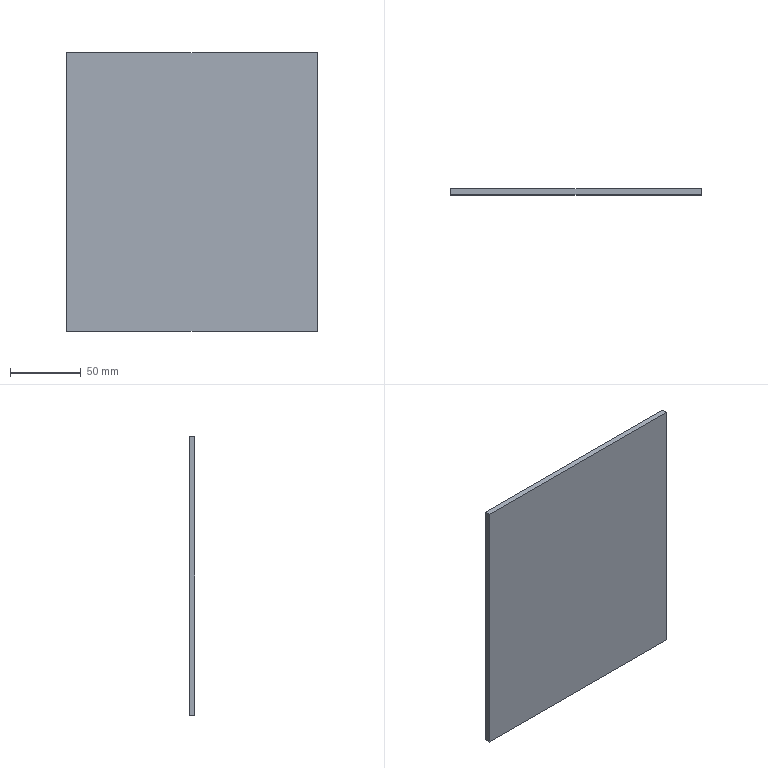Component | SolidWorks | Cover1-5XG1-1 | 1 solid | 6 faces | box 177 x 4 x 197 mm | volume 139476 mm3 | plane 6
build123d program:
from build123d import *

# Parameters (mm, degrees)
SKETCH3_W           = 177
SKETCH3_H           = 197
BOSS_EXTRUDE1_DEPTH = 4


with BuildPart() as part:
    # Sketch3 → Boss-Extrude1 (new body)
    with BuildSketch(Plane.XY):
        Rectangle(SKETCH3_W, SKETCH3_H)
    extrude(amount=BOSS_EXTRUDE1_DEPTH)


solid = part.part

# Placed as in the assembly
solid = solid.moved(Location((0, -154.8, 130), (90, 0, 0)))
STEP:
#1=COLOUR_RGB('',0.7922,0.8196,0.9333);
#2=FILL_AREA_STYLE_COLOUR('',#1);
#3=FILL_AREA_STYLE('',(#2));
#4=SURFACE_STYLE_FILL_AREA(#3);
#5=SURFACE_SIDE_STYLE('',(#4));
#6=SURFACE_STYLE_USAGE(.BOTH.,#5);
#7=PRESENTATION_STYLE_ASSIGNMENT((#6));
#8=CARTESIAN_POINT('',(-3.484,-6.252,1.24));
#9=VERTEX_POINT('',#8);
#10=CARTESIAN_POINT('',(-3.484,-6.252,8.996));
#11=VERTEX_POINT('',#10);
#12=CARTESIAN_POINT('',(-3.484,-6.252,1.24));
#13=DIRECTION('',(-0.,-0.,1.));
#14=VECTOR('',#13,39.37);
#15=LINE('',#12,#14);
#16=EDGE_CURVE('',#9,#11,#15,.T.);
#17=ORIENTED_EDGE('',*,*,#16,.T.);
#18=CARTESIAN_POINT('',(-3.484,-6.094,8.996));
#19=VERTEX_POINT('',#18);
#20=CARTESIAN_POINT('',(-3.484,-6.094,8.996));
#21=DIRECTION('',(-0.,-1.,-0.));
#22=VECTOR('',#21,39.37);
#23=LINE('',#20,#22);
#24=EDGE_CURVE('',#19,#11,#23,.T.);
#25=ORIENTED_EDGE('',*,*,#24,.F.);
#26=CARTESIAN_POINT('',(-3.484,-6.094,1.24));
#27=VERTEX_POINT('',#26);
#28=CARTESIAN_POINT('',(-3.484,-6.094,1.24));
#29=DIRECTION('',(-0.,-0.,1.));
#30=VECTOR('',#29,39.37);
#31=LINE('',#28,#30);
#32=EDGE_CURVE('',#27,#19,#31,.T.);
#33=ORIENTED_EDGE('',*,*,#32,.F.);
#34=CARTESIAN_POINT('',(-3.484,-6.094,1.24));
#35=DIRECTION('',(-0.,-1.,-0.));
#36=VECTOR('',#35,39.37);
#37=LINE('',#34,#36);
#38=EDGE_CURVE('',#27,#9,#37,.T.);
#39=ORIENTED_EDGE('',*,*,#38,.T.);
#40=EDGE_LOOP('',(#17,#25,#33,#39));
#41=FACE_OUTER_BOUND('',#40,.T.);
#42=CARTESIAN_POINT('',(-3.484,-6.094,1.24));
#43=DIRECTION('',(1.,-0.,0.));
#44=DIRECTION('',(-0.,-1.,-0.));
#45=AXIS2_PLACEMENT_3D('',#42,#43,#44);
#46=PLANE('',#45);
#47=ADVANCED_FACE('',(#41),#46,.F.);
#48=CARTESIAN_POINT('',(3.484,-6.252,8.996));
#49=VERTEX_POINT('',#48);
#50=CARTESIAN_POINT('',(-3.484,-6.252,8.996));
#51=DIRECTION('',(1.,-0.,0.));
#52=VECTOR('',#51,39.37);
#53=LINE('',#50,#52);
#54=EDGE_CURVE('',#11,#49,#53,.T.);
#55=ORIENTED_EDGE('',*,*,#54,.T.);
#56=CARTESIAN_POINT('',(3.484,-6.094,8.996));
#57=VERTEX_POINT('',#56);
#58=CARTESIAN_POINT('',(3.484,-6.094,8.996));
#59=DIRECTION('',(-0.,-1.,-0.));
#60=VECTOR('',#59,39.37);
#61=LINE('',#58,#60);
#62=EDGE_CURVE('',#57,#49,#61,.T.);
#63=ORIENTED_EDGE('',*,*,#62,.F.);
#64=CARTESIAN_POINT('',(-3.484,-6.094,8.996));
#65=DIRECTION('',(1.,-0.,0.));
#66=VECTOR('',#65,39.37);
#67=LINE('',#64,#66);
#68=EDGE_CURVE('',#19,#57,#67,.T.);
#69=ORIENTED_EDGE('',*,*,#68,.F.);
#70=ORIENTED_EDGE('',*,*,#24,.T.);
#71=EDGE_LOOP('',(#55,#63,#69,#70));
#72=FACE_OUTER_BOUND('',#71,.T.);
#73=CARTESIAN_POINT('',(-3.484,-6.094,8.996));
#74=DIRECTION('',(0.,0.,-1.));
#75=DIRECTION('',(0.,1.,0.));
#76=AXIS2_PLACEMENT_3D('',#73,#74,#75);
#77=PLANE('',#76);
#78=ADVANCED_FACE('',(#72),#77,.F.);
#79=CARTESIAN_POINT('',(3.484,-6.252,1.24));
#80=VERTEX_POINT('',#79);
#81=CARTESIAN_POINT('',(3.484,-6.252,1.24));
#82=DIRECTION('',(0.,0.,-1.));
#83=VECTOR('',#82,39.37);
#84=LINE('',#81,#83);
#85=EDGE_CURVE('',#49,#80,#84,.T.);
#86=ORIENTED_EDGE('',*,*,#85,.T.);
#87=CARTESIAN_POINT('',(3.484,-6.094,1.24));
#88=VERTEX_POINT('',#87);
#89=CARTESIAN_POINT('',(3.484,-6.094,1.24));
#90=DIRECTION('',(-0.,-1.,-0.));
#91=VECTOR('',#90,39.37);
#92=LINE('',#89,#91);
#93=EDGE_CURVE('',#88,#80,#92,.T.);
#94=ORIENTED_EDGE('',*,*,#93,.F.);
#95=CARTESIAN_POINT('',(3.484,-6.094,1.24));
#96=DIRECTION('',(0.,0.,-1.));
#97=VECTOR('',#96,39.37);
#98=LINE('',#95,#97);
#99=EDGE_CURVE('',#57,#88,#98,.T.);
#100=ORIENTED_EDGE('',*,*,#99,.F.);
#101=ORIENTED_EDGE('',*,*,#62,.T.);
#102=EDGE_LOOP('',(#86,#94,#100,#101));
#103=FACE_OUTER_BOUND('',#102,.T.);
#104=CARTESIAN_POINT('',(3.484,-6.094,1.24));
#105=DIRECTION('',(-1.,0.,-0.));
#106=DIRECTION('',(0.,1.,0.));
#107=AXIS2_PLACEMENT_3D('',#104,#105,#106);
#108=PLANE('',#107);
#109=ADVANCED_FACE('',(#103),#108,.F.);
#110=CARTESIAN_POINT('',(-3.484,-6.252,1.24));
#111=DIRECTION('',(-1.,0.,-0.));
#112=VECTOR('',#111,39.37);
#113=LINE('',#110,#112);
#114=EDGE_CURVE('',#80,#9,#113,.T.);
#115=ORIENTED_EDGE('',*,*,#114,.T.);
#116=ORIENTED_EDGE('',*,*,#38,.F.);
#117=CARTESIAN_POINT('',(-3.484,-6.094,1.24));
#118=DIRECTION('',(-1.,0.,-0.));
#119=VECTOR('',#118,39.37);
#120=LINE('',#117,#119);
#121=EDGE_CURVE('',#88,#27,#120,.T.);
#122=ORIENTED_EDGE('',*,*,#121,.F.);
#123=ORIENTED_EDGE('',*,*,#93,.T.);
#124=EDGE_LOOP('',(#115,#116,#122,#123));
#125=FACE_OUTER_BOUND('',#124,.T.);
#126=CARTESIAN_POINT('',(-3.484,-6.094,1.24));
#127=DIRECTION('',(-0.,-0.,1.));
#128=DIRECTION('',(-0.,-1.,-0.));
#129=AXIS2_PLACEMENT_3D('',#126,#127,#128);
#130=PLANE('',#129);
#131=ADVANCED_FACE('',(#125),#130,.F.);
#132=ORIENTED_EDGE('',*,*,#32,.T.);
#133=ORIENTED_EDGE('',*,*,#68,.T.);
#134=ORIENTED_EDGE('',*,*,#99,.T.);
#135=ORIENTED_EDGE('',*,*,#121,.T.);
#136=EDGE_LOOP('',(#132,#133,#134,#135));
#137=FACE_OUTER_BOUND('',#136,.T.);
#138=CARTESIAN_POINT('',(0.,-6.094,5.118));
#139=DIRECTION('',(0.,1.,0.));
#140=DIRECTION('',(1.,-0.,0.));
#141=AXIS2_PLACEMENT_3D('',#138,#139,#140);
#142=PLANE('',#141);
#143=ADVANCED_FACE('',(#137),#142,.T.);
#144=ORIENTED_EDGE('',*,*,#16,.F.);
#145=ORIENTED_EDGE('',*,*,#114,.F.);
#146=ORIENTED_EDGE('',*,*,#85,.F.);
#147=ORIENTED_EDGE('',*,*,#54,.F.);
#148=EDGE_LOOP('',(#144,#145,#146,#147));
#149=FACE_OUTER_BOUND('',#148,.T.);
#150=CARTESIAN_POINT('',(0.,-6.252,5.118));
#151=DIRECTION('',(0.,1.,0.));
#152=DIRECTION('',(1.,-0.,0.));
#153=AXIS2_PLACEMENT_3D('',#150,#151,#152);
#154=PLANE('',#153);
#155=ADVANCED_FACE('',(#149),#154,.F.);
#156=CLOSED_SHELL('',(#47,#78,#109,#131,#143,#155));
#157=MANIFOLD_SOLID_BREP('',#156);
#158=STYLED_ITEM('',(#7),#157);
#159=(LENGTH_UNIT()NAMED_UNIT(*)SI_UNIT($,.METRE.));
#160=LENGTH_MEASURE_WITH_UNIT(LENGTH_MEASURE(0.0254),#159);
#161=DIMENSIONAL_EXPONENTS(1.,0.,0.,0.,0.,0.,0.);
#162=(CONVERSION_BASED_UNIT('',#160)LENGTH_UNIT()NAMED_UNIT(#161));
#163=UNCERTAINTY_MEASURE_WITH_UNIT(LENGTH_MEASURE(0.00001),#162,'','');
#164=(NAMED_UNIT(*)PLANE_ANGLE_UNIT()SI_UNIT($,.RADIAN.));
#165=(NAMED_UNIT(*)SI_UNIT($,.STERADIAN.)SOLID_ANGLE_UNIT());
#166=(GEOMETRIC_REPRESENTATION_CONTEXT(3)GLOBAL_UNCERTAINTY_ASSIGNED_CONTEXT((#163))GLOBAL_UNIT_ASSIGNED_CONTEXT((#162,#164,#165))REPRESENTATION_CONTEXT('',''));
#167=MECHANICAL_DESIGN_GEOMETRIC_PRESENTATION_REPRESENTATION('',(#158),#166);
#168=CARTESIAN_POINT('',(0.,0.,0.));
#169=DIRECTION('',(0.,0.,1.));
#170=DIRECTION('',(1.,0.,0.));
#171=AXIS2_PLACEMENT_3D('',#168,#169,#170);
#172=(LENGTH_UNIT()NAMED_UNIT(*)SI_UNIT($,.METRE.));
#173=LENGTH_MEASURE_WITH_UNIT(LENGTH_MEASURE(0.0254),#172);
#174=DIMENSIONAL_EXPONENTS(1.,0.,0.,0.,0.,0.,0.);
#175=(CONVERSION_BASED_UNIT('',#173)LENGTH_UNIT()NAMED_UNIT(#174));
#176=UNCERTAINTY_MEASURE_WITH_UNIT(LENGTH_MEASURE(0.00001),#175,'','');
#177=(NAMED_UNIT(*)PLANE_ANGLE_UNIT()SI_UNIT($,.RADIAN.));
#178=(NAMED_UNIT(*)SI_UNIT($,.STERADIAN.)SOLID_ANGLE_UNIT());
#179=(GEOMETRIC_REPRESENTATION_CONTEXT(3)GLOBAL_UNCERTAINTY_ASSIGNED_CONTEXT((#176))GLOBAL_UNIT_ASSIGNED_CONTEXT((#175,#177,#178))REPRESENTATION_CONTEXT('',''));
#180=ADVANCED_BREP_SHAPE_REPRESENTATION('',(#157,#171),#179);
#181=PRESENTATION_LAYER_ASSIGNMENT('','',(#158));